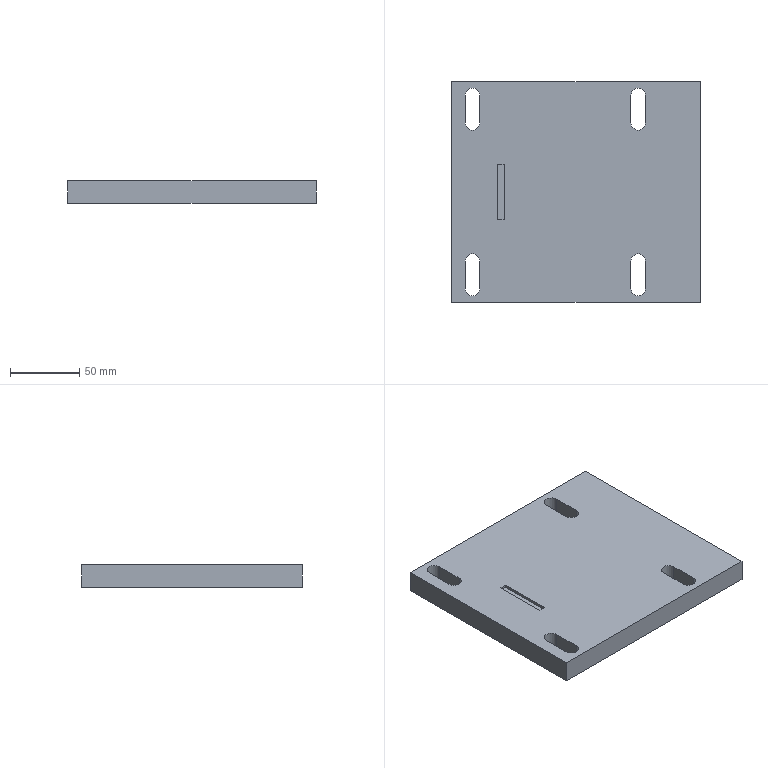Component | SolidWorks | CSFA2082 076-1 | 1 solid | 27 faces | box 180 x 160 x 16 mm | volume 441418 mm3 | plane 19 | cylinder 8 | commonest cylinder face diameters 10.5 x8
build123d program:
from build123d import *

# Parameters (mm, degrees)
SKETCH1_2_W              = 180
SKETCH1_2_H              = 160
EXTRUDE1_DEPTH           = 16
CUT_EXTRUDE1_DEPTH       = 122.474
SKETCH1_W                = 5
SKETCH1_H                = 40
SPRINGCORNERRELIEF_DEPTH = 2


with BuildPart() as part:
    # Sketch1_2 → Extrude1 (new body)
    with BuildSketch(Plane.XY):
        Rectangle(SKETCH1_2_W, SKETCH1_2_H)
    extrude(amount=EXTRUDE1_DEPTH)

    # Sketch2 → Cut-Extrude1 (cut, through all)
    with BuildSketch(Plane.XY.offset(16)):
        with BuildLine():
            Line((-69.75, 70), (-69.75, 50))
            ThreePointArc((-69.75, 50), (-75, 44.75), (-80.25, 50))
            Line((-80.25, 50), (-80.25, 70))
            ThreePointArc((-80.25, 70), (-75, 75.25), (-69.75, 70))
        make_face()
        with BuildLine():
            Line((-69.75, -50), (-69.75, -70))
            ThreePointArc((-69.75, -70), (-75, -75.25), (-80.25, -70))
            Line((-80.25, -70), (-80.25, -50))
            ThreePointArc((-80.25, -50), (-75, -44.75), (-69.75, -50))
        make_face()
        with BuildLine():
            Line((50.25, 70), (50.25, 50))
            ThreePointArc((50.25, 50), (45, 44.75), (39.75, 50))
            Line((39.75, 50), (39.75, 70))
            ThreePointArc((39.75, 70), (45, 75.25), (50.25, 70))
        make_face()
        with BuildLine():
            Line((50.25, -50), (50.25, -70))
            ThreePointArc((50.25, -70), (45, -75.25), (39.75, -70))
            Line((39.75, -70), (39.75, -50))
            ThreePointArc((39.75, -50), (45, -44.75), (50.25, -50))
        make_face()
    extrude(amount=-CUT_EXTRUDE1_DEPTH, mode=Mode.SUBTRACT)

    # Sketch1 → SpringCornerRelief (cut)
    with BuildSketch(Plane.XY.offset(16)):
        with Locations((-54.5, 0)):
            Rectangle(SKETCH1_W, SKETCH1_H)
    extrude(amount=-SPRINGCORNERRELIEF_DEPTH, mode=Mode.SUBTRACT)


solid = part.part

# Placed as in the assembly
solid = solid.moved(Location((187.301, -218.176, 657), (0, 0, 0)))
STEP:
#1=COLOUR_RGB('',0.7922,0.8196,0.9333);
#2=FILL_AREA_STYLE_COLOUR('',#1);
#3=FILL_AREA_STYLE('',(#2));
#4=SURFACE_STYLE_FILL_AREA(#3);
#5=SURFACE_SIDE_STYLE('',(#4));
#6=SURFACE_STYLE_USAGE(.BOTH.,#5);
#7=PRESENTATION_STYLE_ASSIGNMENT((#6));
#8=CARTESIAN_POINT('',(10.917,-11.739,25.866));
#9=VERTEX_POINT('',#8);
#10=CARTESIAN_POINT('',(10.917,-5.44,25.866));
#11=VERTEX_POINT('',#10);
#12=CARTESIAN_POINT('',(10.917,-11.739,25.866));
#13=DIRECTION('',(0.,1.,0.));
#14=VECTOR('',#13,39.37);
#15=LINE('',#12,#14);
#16=EDGE_CURVE('',#9,#11,#15,.T.);
#17=ORIENTED_EDGE('',*,*,#16,.T.);
#18=CARTESIAN_POINT('',(10.917,-5.44,26.496));
#19=VERTEX_POINT('',#18);
#20=CARTESIAN_POINT('',(10.917,-5.44,26.496));
#21=DIRECTION('',(0.,0.,-1.));
#22=VECTOR('',#21,39.37);
#23=LINE('',#20,#22);
#24=EDGE_CURVE('',#19,#11,#23,.T.);
#25=ORIENTED_EDGE('',*,*,#24,.F.);
#26=CARTESIAN_POINT('',(10.917,-11.739,26.496));
#27=VERTEX_POINT('',#26);
#28=CARTESIAN_POINT('',(10.917,-11.739,26.496));
#29=DIRECTION('',(0.,1.,0.));
#30=VECTOR('',#29,39.37);
#31=LINE('',#28,#30);
#32=EDGE_CURVE('',#27,#19,#31,.T.);
#33=ORIENTED_EDGE('',*,*,#32,.F.);
#34=CARTESIAN_POINT('',(10.917,-11.739,26.496));
#35=DIRECTION('',(0.,0.,-1.));
#36=VECTOR('',#35,39.37);
#37=LINE('',#34,#36);
#38=EDGE_CURVE('',#27,#9,#37,.T.);
#39=ORIENTED_EDGE('',*,*,#38,.T.);
#40=EDGE_LOOP('',(#17,#25,#33,#39));
#41=FACE_OUTER_BOUND('',#40,.T.);
#42=CARTESIAN_POINT('',(10.917,-11.739,26.496));
#43=DIRECTION('',(-1.,0.,0.));
#44=DIRECTION('',(0.,0.,1.));
#45=AXIS2_PLACEMENT_3D('',#42,#43,#44);
#46=PLANE('',#45);
#47=ADVANCED_FACE('',(#41),#46,.F.);
#48=CARTESIAN_POINT('',(3.831,-5.44,25.866));
#49=VERTEX_POINT('',#48);
#50=CARTESIAN_POINT('',(3.831,-5.44,25.866));
#51=DIRECTION('',(-1.,0.,0.));
#52=VECTOR('',#51,39.37);
#53=LINE('',#50,#52);
#54=EDGE_CURVE('',#11,#49,#53,.T.);
#55=ORIENTED_EDGE('',*,*,#54,.T.);
#56=CARTESIAN_POINT('',(3.831,-5.44,26.496));
#57=VERTEX_POINT('',#56);
#58=CARTESIAN_POINT('',(3.831,-5.44,26.496));
#59=DIRECTION('',(0.,0.,-1.));
#60=VECTOR('',#59,39.37);
#61=LINE('',#58,#60);
#62=EDGE_CURVE('',#57,#49,#61,.T.);
#63=ORIENTED_EDGE('',*,*,#62,.F.);
#64=CARTESIAN_POINT('',(3.831,-5.44,26.496));
#65=DIRECTION('',(-1.,0.,0.));
#66=VECTOR('',#65,39.37);
#67=LINE('',#64,#66);
#68=EDGE_CURVE('',#19,#57,#67,.T.);
#69=ORIENTED_EDGE('',*,*,#68,.F.);
#70=ORIENTED_EDGE('',*,*,#24,.T.);
#71=EDGE_LOOP('',(#55,#63,#69,#70));
#72=FACE_OUTER_BOUND('',#71,.T.);
#73=CARTESIAN_POINT('',(3.831,-5.44,26.496));
#74=DIRECTION('',(0.,-1.,0.));
#75=DIRECTION('',(0.,0.,-1.));
#76=AXIS2_PLACEMENT_3D('',#73,#74,#75);
#77=PLANE('',#76);
#78=ADVANCED_FACE('',(#72),#77,.F.);
#79=CARTESIAN_POINT('',(3.831,-11.739,25.866));
#80=VERTEX_POINT('',#79);
#81=CARTESIAN_POINT('',(3.831,-11.739,25.866));
#82=DIRECTION('',(0.,-1.,0.));
#83=VECTOR('',#82,39.37);
#84=LINE('',#81,#83);
#85=EDGE_CURVE('',#49,#80,#84,.T.);
#86=ORIENTED_EDGE('',*,*,#85,.T.);
#87=CARTESIAN_POINT('',(3.831,-11.739,26.496));
#88=VERTEX_POINT('',#87);
#89=CARTESIAN_POINT('',(3.831,-11.739,26.496));
#90=DIRECTION('',(0.,0.,-1.));
#91=VECTOR('',#90,39.37);
#92=LINE('',#89,#91);
#93=EDGE_CURVE('',#88,#80,#92,.T.);
#94=ORIENTED_EDGE('',*,*,#93,.F.);
#95=CARTESIAN_POINT('',(3.831,-11.739,26.496));
#96=DIRECTION('',(0.,-1.,0.));
#97=VECTOR('',#96,39.37);
#98=LINE('',#95,#97);
#99=EDGE_CURVE('',#57,#88,#98,.T.);
#100=ORIENTED_EDGE('',*,*,#99,.F.);
#101=ORIENTED_EDGE('',*,*,#62,.T.);
#102=EDGE_LOOP('',(#86,#94,#100,#101));
#103=FACE_OUTER_BOUND('',#102,.T.);
#104=CARTESIAN_POINT('',(3.831,-11.739,26.496));
#105=DIRECTION('',(1.,0.,0.));
#106=DIRECTION('',(0.,0.,-1.));
#107=AXIS2_PLACEMENT_3D('',#104,#105,#106);
#108=PLANE('',#107);
#109=ADVANCED_FACE('',(#103),#108,.F.);
#110=CARTESIAN_POINT('',(3.831,-11.739,25.866));
#111=DIRECTION('',(1.,0.,0.));
#112=VECTOR('',#111,39.37);
#113=LINE('',#110,#112);
#114=EDGE_CURVE('',#80,#9,#113,.T.);
#115=ORIENTED_EDGE('',*,*,#114,.T.);
#116=ORIENTED_EDGE('',*,*,#38,.F.);
#117=CARTESIAN_POINT('',(3.831,-11.739,26.496));
#118=DIRECTION('',(1.,0.,0.));
#119=VECTOR('',#118,39.37);
#120=LINE('',#117,#119);
#121=EDGE_CURVE('',#88,#27,#120,.T.);
#122=ORIENTED_EDGE('',*,*,#121,.F.);
#123=ORIENTED_EDGE('',*,*,#93,.T.);
#124=EDGE_LOOP('',(#115,#116,#122,#123));
#125=FACE_OUTER_BOUND('',#124,.T.);
#126=CARTESIAN_POINT('',(3.831,-11.739,26.496));
#127=DIRECTION('',(0.,1.,0.));
#128=DIRECTION('',(0.,0.,1.));
#129=AXIS2_PLACEMENT_3D('',#126,#127,#128);
#130=PLANE('',#129);
#131=ADVANCED_FACE('',(#125),#130,.F.);
#132=CARTESIAN_POINT('',(5.13,-9.377,26.496));
#133=VERTEX_POINT('',#132);
#134=CARTESIAN_POINT('',(5.327,-9.377,26.496));
#135=VERTEX_POINT('',#134);
#136=CARTESIAN_POINT('',(5.13,-9.377,26.496));
#137=DIRECTION('',(1.,0.,0.));
#138=VECTOR('',#137,39.37);
#139=LINE('',#136,#138);
#140=EDGE_CURVE('',#133,#135,#139,.T.);
#141=ORIENTED_EDGE('',*,*,#140,.F.);
#142=CARTESIAN_POINT('',(5.13,-7.802,26.496));
#143=VERTEX_POINT('',#142);
#144=CARTESIAN_POINT('',(5.13,-9.377,26.496));
#145=DIRECTION('',(0.,-1.,0.));
#146=VECTOR('',#145,39.37);
#147=LINE('',#144,#146);
#148=EDGE_CURVE('',#143,#133,#147,.T.);
#149=ORIENTED_EDGE('',*,*,#148,.F.);
#150=CARTESIAN_POINT('',(5.327,-7.802,26.496));
#151=VERTEX_POINT('',#150);
#152=CARTESIAN_POINT('',(5.13,-7.802,26.496));
#153=DIRECTION('',(-1.,0.,0.));
#154=VECTOR('',#153,39.37);
#155=LINE('',#152,#154);
#156=EDGE_CURVE('',#151,#143,#155,.T.);
#157=ORIENTED_EDGE('',*,*,#156,.F.);
#158=CARTESIAN_POINT('',(5.327,-9.377,26.496));
#159=DIRECTION('',(0.,1.,0.));
#160=VECTOR('',#159,39.37);
#161=LINE('',#158,#160);
#162=EDGE_CURVE('',#135,#151,#161,.T.);
#163=ORIENTED_EDGE('',*,*,#162,.F.);
#164=EDGE_LOOP('',(#141,#149,#157,#163));
#165=FACE_BOUND('',#164,.T.);
#166=CARTESIAN_POINT('',(8.939,-10.558,26.496));
#167=VERTEX_POINT('',#166);
#168=CARTESIAN_POINT('',(8.939,-11.346,26.496));
#169=VERTEX_POINT('',#168);
#170=CARTESIAN_POINT('',(8.939,-10.558,26.496));
#171=DIRECTION('',(0.,-1.,0.));
#172=VECTOR('',#171,39.37);
#173=LINE('',#170,#172);
#174=EDGE_CURVE('',#167,#169,#173,.T.);
#175=ORIENTED_EDGE('',*,*,#174,.F.);
#176=CARTESIAN_POINT('',(9.352,-10.558,26.496));
#177=VERTEX_POINT('',#176);
#178=CARTESIAN_POINT('',(9.146,-10.558,26.496));
#179=DIRECTION('',(0.,0.,1.));
#180=DIRECTION('',(1.,0.,0.));
#181=AXIS2_PLACEMENT_3D('',#178,#179,#180);
#182=CIRCLE('',#181,0.2067);
#183=EDGE_CURVE('',#177,#167,#182,.T.);
#184=ORIENTED_EDGE('',*,*,#183,.F.);
#185=CARTESIAN_POINT('',(9.352,-11.346,26.496));
#186=VERTEX_POINT('',#185);
#187=CARTESIAN_POINT('',(9.352,-10.558,26.496));
#188=DIRECTION('',(0.,1.,0.));
#189=VECTOR('',#188,39.37);
#190=LINE('',#187,#189);
#191=EDGE_CURVE('',#186,#177,#190,.T.);
#192=ORIENTED_EDGE('',*,*,#191,.F.);
#193=CARTESIAN_POINT('',(9.146,-11.346,26.496));
#194=DIRECTION('',(0.,0.,1.));
#195=DIRECTION('',(1.,0.,0.));
#196=AXIS2_PLACEMENT_3D('',#193,#194,#195);
#197=CIRCLE('',#196,0.2067);
#198=EDGE_CURVE('',#169,#186,#197,.T.);
#199=ORIENTED_EDGE('',*,*,#198,.F.);
#200=EDGE_LOOP('',(#175,#184,#192,#199));
#201=FACE_BOUND('',#200,.T.);
#202=CARTESIAN_POINT('',(8.939,-5.834,26.496));
#203=VERTEX_POINT('',#202);
#204=CARTESIAN_POINT('',(8.939,-6.621,26.496));
#205=VERTEX_POINT('',#204);
#206=CARTESIAN_POINT('',(8.939,-5.834,26.496));
#207=DIRECTION('',(0.,-1.,0.));
#208=VECTOR('',#207,39.37);
#209=LINE('',#206,#208);
#210=EDGE_CURVE('',#203,#205,#209,.T.);
#211=ORIENTED_EDGE('',*,*,#210,.F.);
#212=CARTESIAN_POINT('',(9.352,-5.834,26.496));
#213=VERTEX_POINT('',#212);
#214=CARTESIAN_POINT('',(9.146,-5.834,26.496));
#215=DIRECTION('',(0.,0.,1.));
#216=DIRECTION('',(1.,0.,0.));
#217=AXIS2_PLACEMENT_3D('',#214,#215,#216);
#218=CIRCLE('',#217,0.2067);
#219=EDGE_CURVE('',#213,#203,#218,.T.);
#220=ORIENTED_EDGE('',*,*,#219,.F.);
#221=CARTESIAN_POINT('',(9.352,-6.621,26.496));
#222=VERTEX_POINT('',#221);
#223=CARTESIAN_POINT('',(9.352,-5.834,26.496));
#224=DIRECTION('',(0.,1.,0.));
#225=VECTOR('',#224,39.37);
#226=LINE('',#223,#225);
#227=EDGE_CURVE('',#222,#213,#226,.T.);
#228=ORIENTED_EDGE('',*,*,#227,.F.);
#229=CARTESIAN_POINT('',(9.146,-6.621,26.496));
#230=DIRECTION('',(0.,0.,1.));
#231=DIRECTION('',(1.,0.,0.));
#232=AXIS2_PLACEMENT_3D('',#229,#230,#231);
#233=CIRCLE('',#232,0.2067);
#234=EDGE_CURVE('',#205,#222,#233,.T.);
#235=ORIENTED_EDGE('',*,*,#234,.F.);
#236=EDGE_LOOP('',(#211,#220,#228,#235));
#237=FACE_BOUND('',#236,.T.);
#238=CARTESIAN_POINT('',(4.215,-10.558,26.496));
#239=VERTEX_POINT('',#238);
#240=CARTESIAN_POINT('',(4.215,-11.346,26.496));
#241=VERTEX_POINT('',#240);
#242=CARTESIAN_POINT('',(4.215,-10.558,26.496));
#243=DIRECTION('',(0.,-1.,0.));
#244=VECTOR('',#243,39.37);
#245=LINE('',#242,#244);
#246=EDGE_CURVE('',#239,#241,#245,.T.);
#247=ORIENTED_EDGE('',*,*,#246,.F.);
#248=CARTESIAN_POINT('',(4.628,-10.558,26.496));
#249=VERTEX_POINT('',#248);
#250=CARTESIAN_POINT('',(4.421,-10.558,26.496));
#251=DIRECTION('',(0.,0.,1.));
#252=DIRECTION('',(1.,0.,0.));
#253=AXIS2_PLACEMENT_3D('',#250,#251,#252);
#254=CIRCLE('',#253,0.2067);
#255=EDGE_CURVE('',#249,#239,#254,.T.);
#256=ORIENTED_EDGE('',*,*,#255,.F.);
#257=CARTESIAN_POINT('',(4.628,-11.346,26.496));
#258=VERTEX_POINT('',#257);
#259=CARTESIAN_POINT('',(4.628,-10.558,26.496));
#260=DIRECTION('',(0.,1.,0.));
#261=VECTOR('',#260,39.37);
#262=LINE('',#259,#261);
#263=EDGE_CURVE('',#258,#249,#262,.T.);
#264=ORIENTED_EDGE('',*,*,#263,.F.);
#265=CARTESIAN_POINT('',(4.421,-11.346,26.496));
#266=DIRECTION('',(0.,0.,1.));
#267=DIRECTION('',(1.,0.,0.));
#268=AXIS2_PLACEMENT_3D('',#265,#266,#267);
#269=CIRCLE('',#268,0.2067);
#270=EDGE_CURVE('',#241,#258,#269,.T.);
#271=ORIENTED_EDGE('',*,*,#270,.F.);
#272=EDGE_LOOP('',(#247,#256,#264,#271));
#273=FACE_BOUND('',#272,.T.);
#274=CARTESIAN_POINT('',(4.215,-5.834,26.496));
#275=VERTEX_POINT('',#274);
#276=CARTESIAN_POINT('',(4.215,-6.621,26.496));
#277=VERTEX_POINT('',#276);
#278=CARTESIAN_POINT('',(4.215,-5.834,26.496));
#279=DIRECTION('',(0.,-1.,0.));
#280=VECTOR('',#279,39.37);
#281=LINE('',#278,#280);
#282=EDGE_CURVE('',#275,#277,#281,.T.);
#283=ORIENTED_EDGE('',*,*,#282,.F.);
#284=CARTESIAN_POINT('',(4.628,-5.834,26.496));
#285=VERTEX_POINT('',#284);
#286=CARTESIAN_POINT('',(4.421,-5.834,26.496));
#287=DIRECTION('',(0.,0.,1.));
#288=DIRECTION('',(1.,0.,0.));
#289=AXIS2_PLACEMENT_3D('',#286,#287,#288);
#290=CIRCLE('',#289,0.2067);
#291=EDGE_CURVE('',#285,#275,#290,.T.);
#292=ORIENTED_EDGE('',*,*,#291,.F.);
#293=CARTESIAN_POINT('',(4.628,-6.621,26.496));
#294=VERTEX_POINT('',#293);
#295=CARTESIAN_POINT('',(4.628,-5.834,26.496));
#296=DIRECTION('',(0.,1.,0.));
#297=VECTOR('',#296,39.37);
#298=LINE('',#295,#297);
#299=EDGE_CURVE('',#294,#285,#298,.T.);
#300=ORIENTED_EDGE('',*,*,#299,.F.);
#301=CARTESIAN_POINT('',(4.421,-6.621,26.496));
#302=DIRECTION('',(0.,0.,1.));
#303=DIRECTION('',(1.,0.,0.));
#304=AXIS2_PLACEMENT_3D('',#301,#302,#303);
#305=CIRCLE('',#304,0.2067);
#306=EDGE_CURVE('',#277,#294,#305,.T.);
#307=ORIENTED_EDGE('',*,*,#306,.F.);
#308=EDGE_LOOP('',(#283,#292,#300,#307));
#309=FACE_BOUND('',#308,.T.);
#310=ORIENTED_EDGE('',*,*,#32,.T.);
#311=ORIENTED_EDGE('',*,*,#68,.T.);
#312=ORIENTED_EDGE('',*,*,#99,.T.);
#313=ORIENTED_EDGE('',*,*,#121,.T.);
#314=EDGE_LOOP('',(#310,#311,#312,#313));
#315=FACE_OUTER_BOUND('',#314,.T.);
#316=CARTESIAN_POINT('',(10.917,-5.44,26.496));
#317=DIRECTION('',(0.,0.,-1.));
#318=DIRECTION('',(-1.,0.,0.));
#319=AXIS2_PLACEMENT_3D('',#316,#317,#318);
#320=PLANE('',#319);
#321=ADVANCED_FACE('',(#165,#201,#237,#273,#309,#315),#320,.F.);
#322=CARTESIAN_POINT('',(9.352,-10.558,25.866));
#323=VERTEX_POINT('',#322);
#324=CARTESIAN_POINT('',(8.939,-10.558,25.866));
#325=VERTEX_POINT('',#324);
#326=CARTESIAN_POINT('',(9.146,-10.558,25.866));
#327=DIRECTION('',(0.,0.,1.));
#328=DIRECTION('',(1.,0.,0.));
#329=AXIS2_PLACEMENT_3D('',#326,#327,#328);
#330=CIRCLE('',#329,0.2067);
#331=EDGE_CURVE('',#323,#325,#330,.T.);
#332=ORIENTED_EDGE('',*,*,#331,.T.);
#333=CARTESIAN_POINT('',(8.939,-11.346,25.866));
#334=VERTEX_POINT('',#333);
#335=CARTESIAN_POINT('',(8.939,-10.558,25.866));
#336=DIRECTION('',(0.,-1.,0.));
#337=VECTOR('',#336,39.37);
#338=LINE('',#335,#337);
#339=EDGE_CURVE('',#325,#334,#338,.T.);
#340=ORIENTED_EDGE('',*,*,#339,.T.);
#341=CARTESIAN_POINT('',(9.352,-11.346,25.866));
#342=VERTEX_POINT('',#341);
#343=CARTESIAN_POINT('',(9.146,-11.346,25.866));
#344=DIRECTION('',(0.,0.,1.));
#345=DIRECTION('',(1.,0.,0.));
#346=AXIS2_PLACEMENT_3D('',#343,#344,#345);
#347=CIRCLE('',#346,0.2067);
#348=EDGE_CURVE('',#334,#342,#347,.T.);
#349=ORIENTED_EDGE('',*,*,#348,.T.);
#350=CARTESIAN_POINT('',(9.352,-10.558,25.866));
#351=DIRECTION('',(0.,1.,0.));
#352=VECTOR('',#351,39.37);
#353=LINE('',#350,#352);
#354=EDGE_CURVE('',#342,#323,#353,.T.);
#355=ORIENTED_EDGE('',*,*,#354,.T.);
#356=EDGE_LOOP('',(#332,#340,#349,#355));
#357=FACE_BOUND('',#356,.T.);
#358=CARTESIAN_POINT('',(9.352,-5.834,25.866));
#359=VERTEX_POINT('',#358);
#360=CARTESIAN_POINT('',(8.939,-5.834,25.866));
#361=VERTEX_POINT('',#360);
#362=CARTESIAN_POINT('',(9.146,-5.834,25.866));
#363=DIRECTION('',(0.,0.,1.));
#364=DIRECTION('',(1.,0.,0.));
#365=AXIS2_PLACEMENT_3D('',#362,#363,#364);
#366=CIRCLE('',#365,0.2067);
#367=EDGE_CURVE('',#359,#361,#366,.T.);
#368=ORIENTED_EDGE('',*,*,#367,.T.);
#369=CARTESIAN_POINT('',(8.939,-6.621,25.866));
#370=VERTEX_POINT('',#369);
#371=CARTESIAN_POINT('',(8.939,-5.834,25.866));
#372=DIRECTION('',(0.,-1.,0.));
#373=VECTOR('',#372,39.37);
#374=LINE('',#371,#373);
#375=EDGE_CURVE('',#361,#370,#374,.T.);
#376=ORIENTED_EDGE('',*,*,#375,.T.);
#377=CARTESIAN_POINT('',(9.352,-6.621,25.866));
#378=VERTEX_POINT('',#377);
#379=CARTESIAN_POINT('',(9.146,-6.621,25.866));
#380=DIRECTION('',(0.,0.,1.));
#381=DIRECTION('',(1.,0.,0.));
#382=AXIS2_PLACEMENT_3D('',#379,#380,#381);
#383=CIRCLE('',#382,0.2067);
#384=EDGE_CURVE('',#370,#378,#383,.T.);
#385=ORIENTED_EDGE('',*,*,#384,.T.);
#386=CARTESIAN_POINT('',(9.352,-5.834,25.866));
#387=DIRECTION('',(0.,1.,0.));
#388=VECTOR('',#387,39.37);
#389=LINE('',#386,#388);
#390=EDGE_CURVE('',#378,#359,#389,.T.);
#391=ORIENTED_EDGE('',*,*,#390,.T.);
#392=EDGE_LOOP('',(#368,#376,#385,#391));
#393=FACE_BOUND('',#392,.T.);
#394=CARTESIAN_POINT('',(4.628,-10.558,25.866));
#395=VERTEX_POINT('',#394);
#396=CARTESIAN_POINT('',(4.215,-10.558,25.866));
#397=VERTEX_POINT('',#396);
#398=CARTESIAN_POINT('',(4.421,-10.558,25.866));
#399=DIRECTION('',(0.,0.,1.));
#400=DIRECTION('',(1.,0.,0.));
#401=AXIS2_PLACEMENT_3D('',#398,#399,#400);
#402=CIRCLE('',#401,0.2067);
#403=EDGE_CURVE('',#395,#397,#402,.T.);
#404=ORIENTED_EDGE('',*,*,#403,.T.);
#405=CARTESIAN_POINT('',(4.215,-11.346,25.866));
#406=VERTEX_POINT('',#405);
#407=CARTESIAN_POINT('',(4.215,-10.558,25.866));
#408=DIRECTION('',(0.,-1.,0.));
#409=VECTOR('',#408,39.37);
#410=LINE('',#407,#409);
#411=EDGE_CURVE('',#397,#406,#410,.T.);
#412=ORIENTED_EDGE('',*,*,#411,.T.);
#413=CARTESIAN_POINT('',(4.628,-11.346,25.866));
#414=VERTEX_POINT('',#413);
#415=CARTESIAN_POINT('',(4.421,-11.346,25.866));
#416=DIRECTION('',(0.,0.,1.));
#417=DIRECTION('',(1.,0.,0.));
#418=AXIS2_PLACEMENT_3D('',#415,#416,#417);
#419=CIRCLE('',#418,0.2067);
#420=EDGE_CURVE('',#406,#414,#419,.T.);
#421=ORIENTED_EDGE('',*,*,#420,.T.);
#422=CARTESIAN_POINT('',(4.628,-10.558,25.866));
#423=DIRECTION('',(0.,1.,0.));
#424=VECTOR('',#423,39.37);
#425=LINE('',#422,#424);
#426=EDGE_CURVE('',#414,#395,#425,.T.);
#427=ORIENTED_EDGE('',*,*,#426,.T.);
#428=EDGE_LOOP('',(#404,#412,#421,#427));
#429=FACE_BOUND('',#428,.T.);
#430=CARTESIAN_POINT('',(4.628,-5.834,25.866));
#431=VERTEX_POINT('',#430);
#432=CARTESIAN_POINT('',(4.215,-5.834,25.866));
#433=VERTEX_POINT('',#432);
#434=CARTESIAN_POINT('',(4.421,-5.834,25.866));
#435=DIRECTION('',(0.,0.,1.));
#436=DIRECTION('',(1.,0.,0.));
#437=AXIS2_PLACEMENT_3D('',#434,#435,#436);
#438=CIRCLE('',#437,0.2067);
#439=EDGE_CURVE('',#431,#433,#438,.T.);
#440=ORIENTED_EDGE('',*,*,#439,.T.);
#441=CARTESIAN_POINT('',(4.215,-6.621,25.866));
#442=VERTEX_POINT('',#441);
#443=CARTESIAN_POINT('',(4.215,-5.834,25.866));
#444=DIRECTION('',(0.,-1.,0.));
#445=VECTOR('',#444,39.37);
#446=LINE('',#443,#445);
#447=EDGE_CURVE('',#433,#442,#446,.T.);
#448=ORIENTED_EDGE('',*,*,#447,.T.);
#449=CARTESIAN_POINT('',(4.628,-6.621,25.866));
#450=VERTEX_POINT('',#449);
#451=CARTESIAN_POINT('',(4.421,-6.621,25.866));
#452=DIRECTION('',(0.,0.,1.));
#453=DIRECTION('',(1.,0.,0.));
#454=AXIS2_PLACEMENT_3D('',#451,#452,#453);
#455=CIRCLE('',#454,0.2067);
#456=EDGE_CURVE('',#442,#450,#455,.T.);
#457=ORIENTED_EDGE('',*,*,#456,.T.);
#458=CARTESIAN_POINT('',(4.628,-5.834,25.866));
#459=DIRECTION('',(0.,1.,0.));
#460=VECTOR('',#459,39.37);
#461=LINE('',#458,#460);
#462=EDGE_CURVE('',#450,#431,#461,.T.);
#463=ORIENTED_EDGE('',*,*,#462,.T.);
#464=EDGE_LOOP('',(#440,#448,#457,#463));
#465=FACE_BOUND('',#464,.T.);
#466=ORIENTED_EDGE('',*,*,#16,.F.);
#467=ORIENTED_EDGE('',*,*,#114,.F.);
#468=ORIENTED_EDGE('',*,*,#85,.F.);
#469=ORIENTED_EDGE('',*,*,#54,.F.);
#470=EDGE_LOOP('',(#466,#467,#468,#469));
#471=FACE_OUTER_BOUND('',#470,.T.);
#472=CARTESIAN_POINT('',(10.917,-5.44,25.866));
#473=DIRECTION('',(0.,0.,-1.));
#474=DIRECTION('',(-1.,0.,0.));
#475=AXIS2_PLACEMENT_3D('',#472,#473,#474);
#476=PLANE('',#475);
#477=ADVANCED_FACE('',(#357,#393,#429,#465,#471),#476,.T.);
#478=ORIENTED_EDGE('',*,*,#291,.T.);
#479=CARTESIAN_POINT('',(4.215,-5.834,25.866));
#480=DIRECTION('',(0.,0.,1.));
#481=VECTOR('',#480,39.37);
#482=LINE('',#479,#481);
#483=EDGE_CURVE('',#433,#275,#482,.T.);
#484=ORIENTED_EDGE('',*,*,#483,.F.);
#485=ORIENTED_EDGE('',*,*,#439,.F.);
#486=CARTESIAN_POINT('',(4.628,-5.834,25.866));
#487=DIRECTION('',(0.,0.,1.));
#488=VECTOR('',#487,39.37);
#489=LINE('',#486,#488);
#490=EDGE_CURVE('',#431,#285,#489,.T.);
#491=ORIENTED_EDGE('',*,*,#490,.T.);
#492=EDGE_LOOP('',(#478,#484,#485,#491));
#493=FACE_OUTER_BOUND('',#492,.T.);
#494=CARTESIAN_POINT('',(4.421,-5.834,25.866));
#495=DIRECTION('',(0.,0.,1.));
#496=DIRECTION('',(1.,0.,0.));
#497=AXIS2_PLACEMENT_3D('',#494,#495,#496);
#498=CYLINDRICAL_SURFACE('',#497,0.2067);
#499=ADVANCED_FACE('',(#493),#498,.F.);
#500=ORIENTED_EDGE('',*,*,#299,.T.);
#501=ORIENTED_EDGE('',*,*,#490,.F.);
#502=ORIENTED_EDGE('',*,*,#462,.F.);
#503=CARTESIAN_POINT('',(4.628,-6.621,25.866));
#504=DIRECTION('',(0.,0.,1.));
#505=VECTOR('',#504,39.37);
#506=LINE('',#503,#505);
#507=EDGE_CURVE('',#450,#294,#506,.T.);
#508=ORIENTED_EDGE('',*,*,#507,.T.);
#509=EDGE_LOOP('',(#500,#501,#502,#508));
#510=FACE_OUTER_BOUND('',#509,.T.);
#511=CARTESIAN_POINT('',(4.628,-5.834,25.866));
#512=DIRECTION('',(1.,0.,0.));
#513=DIRECTION('',(0.,0.,-1.));
#514=AXIS2_PLACEMENT_3D('',#511,#512,#513);
#515=PLANE('',#514);
#516=ADVANCED_FACE('',(#510),#515,.F.);
#517=ORIENTED_EDGE('',*,*,#306,.T.);
#518=ORIENTED_EDGE('',*,*,#507,.F.);
#519=ORIENTED_EDGE('',*,*,#456,.F.);
#520=CARTESIAN_POINT('',(4.215,-6.621,25.866));
#521=DIRECTION('',(0.,0.,1.));
#522=VECTOR('',#521,39.37);
#523=LINE('',#520,#522);
#524=EDGE_CURVE('',#442,#277,#523,.T.);
#525=ORIENTED_EDGE('',*,*,#524,.T.);
#526=EDGE_LOOP('',(#517,#518,#519,#525));
#527=FACE_OUTER_BOUND('',#526,.T.);
#528=CARTESIAN_POINT('',(4.421,-6.621,25.866));
#529=DIRECTION('',(0.,0.,1.));
#530=DIRECTION('',(1.,0.,0.));
#531=AXIS2_PLACEMENT_3D('',#528,#529,#530);
#532=CYLINDRICAL_SURFACE('',#531,0.2067);
#533=ADVANCED_FACE('',(#527),#532,.F.);
#534=ORIENTED_EDGE('',*,*,#282,.T.);
#535=ORIENTED_EDGE('',*,*,#524,.F.);
#536=ORIENTED_EDGE('',*,*,#447,.F.);
#537=ORIENTED_EDGE('',*,*,#483,.T.);
#538=EDGE_LOOP('',(#534,#535,#536,#537));
#539=FACE_OUTER_BOUND('',#538,.T.);
#540=CARTESIAN_POINT('',(4.215,-5.834,25.866));
#541=DIRECTION('',(-1.,0.,0.));
#542=DIRECTION('',(0.,0.,1.));
#543=AXIS2_PLACEMENT_3D('',#540,#541,#542);
#544=PLANE('',#543);
#545=ADVANCED_FACE('',(#539),#544,.F.);
#546=ORIENTED_EDGE('',*,*,#255,.T.);
#547=CARTESIAN_POINT('',(4.215,-10.558,25.866));
#548=DIRECTION('',(0.,0.,1.));
#549=VECTOR('',#548,39.37);
#550=LINE('',#547,#549);
#551=EDGE_CURVE('',#397,#239,#550,.T.);
#552=ORIENTED_EDGE('',*,*,#551,.F.);
#553=ORIENTED_EDGE('',*,*,#403,.F.);
#554=CARTESIAN_POINT('',(4.628,-10.558,25.866));
#555=DIRECTION('',(0.,0.,1.));
#556=VECTOR('',#555,39.37);
#557=LINE('',#554,#556);
#558=EDGE_CURVE('',#395,#249,#557,.T.);
#559=ORIENTED_EDGE('',*,*,#558,.T.);
#560=EDGE_LOOP('',(#546,#552,#553,#559));
#561=FACE_OUTER_BOUND('',#560,.T.);
#562=CARTESIAN_POINT('',(4.421,-10.558,25.866));
#563=DIRECTION('',(0.,0.,1.));
#564=DIRECTION('',(1.,0.,0.));
#565=AXIS2_PLACEMENT_3D('',#562,#563,#564);
#566=CYLINDRICAL_SURFACE('',#565,0.2067);
#567=ADVANCED_FACE('',(#561),#566,.F.);
#568=ORIENTED_EDGE('',*,*,#263,.T.);
#569=ORIENTED_EDGE('',*,*,#558,.F.);
#570=ORIENTED_EDGE('',*,*,#426,.F.);
#571=CARTESIAN_POINT('',(4.628,-11.346,25.866));
#572=DIRECTION('',(0.,0.,1.));
#573=VECTOR('',#572,39.37);
#574=LINE('',#571,#573);
#575=EDGE_CURVE('',#414,#258,#574,.T.);
#576=ORIENTED_EDGE('',*,*,#575,.T.);
#577=EDGE_LOOP('',(#568,#569,#570,#576));
#578=FACE_OUTER_BOUND('',#577,.T.);
#579=CARTESIAN_POINT('',(4.628,-10.558,25.866));
#580=DIRECTION('',(1.,0.,0.));
#581=DIRECTION('',(0.,0.,-1.));
#582=AXIS2_PLACEMENT_3D('',#579,#580,#581);
#583=PLANE('',#582);
#584=ADVANCED_FACE('',(#578),#583,.F.);
#585=ORIENTED_EDGE('',*,*,#270,.T.);
#586=ORIENTED_EDGE('',*,*,#575,.F.);
#587=ORIENTED_EDGE('',*,*,#420,.F.);
#588=CARTESIAN_POINT('',(4.215,-11.346,25.866));
#589=DIRECTION('',(0.,0.,1.));
#590=VECTOR('',#589,39.37);
#591=LINE('',#588,#590);
#592=EDGE_CURVE('',#406,#241,#591,.T.);
#593=ORIENTED_EDGE('',*,*,#592,.T.);
#594=EDGE_LOOP('',(#585,#586,#587,#593));
#595=FACE_OUTER_BOUND('',#594,.T.);
#596=CARTESIAN_POINT('',(4.421,-11.346,25.866));
#597=DIRECTION('',(0.,0.,1.));
#598=DIRECTION('',(1.,0.,0.));
#599=AXIS2_PLACEMENT_3D('',#596,#597,#598);
#600=CYLINDRICAL_SURFACE('',#599,0.2067);
#601=ADVANCED_FACE('',(#595),#600,.F.);
#602=ORIENTED_EDGE('',*,*,#246,.T.);
#603=ORIENTED_EDGE('',*,*,#592,.F.);
#604=ORIENTED_EDGE('',*,*,#411,.F.);
#605=ORIENTED_EDGE('',*,*,#551,.T.);
#606=EDGE_LOOP('',(#602,#603,#604,#605));
#607=FACE_OUTER_BOUND('',#606,.T.);
#608=CARTESIAN_POINT('',(4.215,-10.558,25.866));
#609=DIRECTION('',(-1.,0.,0.));
#610=DIRECTION('',(0.,0.,1.));
#611=AXIS2_PLACEMENT_3D('',#608,#609,#610);
#612=PLANE('',#611);
#613=ADVANCED_FACE('',(#607),#612,.F.);
#614=ORIENTED_EDGE('',*,*,#219,.T.);
#615=CARTESIAN_POINT('',(8.939,-5.834,25.866));
#616=DIRECTION('',(0.,0.,1.));
#617=VECTOR('',#616,39.37);
#618=LINE('',#615,#617);
#619=EDGE_CURVE('',#361,#203,#618,.T.);
#620=ORIENTED_EDGE('',*,*,#619,.F.);
#621=ORIENTED_EDGE('',*,*,#367,.F.);
#622=CARTESIAN_POINT('',(9.352,-5.834,25.866));
#623=DIRECTION('',(0.,0.,1.));
#624=VECTOR('',#623,39.37);
#625=LINE('',#622,#624);
#626=EDGE_CURVE('',#359,#213,#625,.T.);
#627=ORIENTED_EDGE('',*,*,#626,.T.);
#628=EDGE_LOOP('',(#614,#620,#621,#627));
#629=FACE_OUTER_BOUND('',#628,.T.);
#630=CARTESIAN_POINT('',(9.146,-5.834,25.866));
#631=DIRECTION('',(0.,0.,1.));
#632=DIRECTION('',(1.,0.,0.));
#633=AXIS2_PLACEMENT_3D('',#630,#631,#632);
#634=CYLINDRICAL_SURFACE('',#633,0.2067);
#635=ADVANCED_FACE('',(#629),#634,.F.);
#636=ORIENTED_EDGE('',*,*,#227,.T.);
#637=ORIENTED_EDGE('',*,*,#626,.F.);
#638=ORIENTED_EDGE('',*,*,#390,.F.);
#639=CARTESIAN_POINT('',(9.352,-6.621,25.866));
#640=DIRECTION('',(0.,0.,1.));
#641=VECTOR('',#640,39.37);
#642=LINE('',#639,#641);
#643=EDGE_CURVE('',#378,#222,#642,.T.);
#644=ORIENTED_EDGE('',*,*,#643,.T.);
#645=EDGE_LOOP('',(#636,#637,#638,#644));
#646=FACE_OUTER_BOUND('',#645,.T.);
#647=CARTESIAN_POINT('',(9.352,-5.834,25.866));
#648=DIRECTION('',(1.,0.,0.));
#649=DIRECTION('',(0.,0.,-1.));
#650=AXIS2_PLACEMENT_3D('',#647,#648,#649);
#651=PLANE('',#650);
#652=ADVANCED_FACE('',(#646),#651,.F.);
#653=ORIENTED_EDGE('',*,*,#234,.T.);
#654=ORIENTED_EDGE('',*,*,#643,.F.);
#655=ORIENTED_EDGE('',*,*,#384,.F.);
#656=CARTESIAN_POINT('',(8.939,-6.621,25.866));
#657=DIRECTION('',(0.,0.,1.));
#658=VECTOR('',#657,39.37);
#659=LINE('',#656,#658);
#660=EDGE_CURVE('',#370,#205,#659,.T.);
#661=ORIENTED_EDGE('',*,*,#660,.T.);
#662=EDGE_LOOP('',(#653,#654,#655,#661));
#663=FACE_OUTER_BOUND('',#662,.T.);
#664=CARTESIAN_POINT('',(9.146,-6.621,25.866));
#665=DIRECTION('',(0.,0.,1.));
#666=DIRECTION('',(1.,0.,0.));
#667=AXIS2_PLACEMENT_3D('',#664,#665,#666);
#668=CYLINDRICAL_SURFACE('',#667,0.2067);
#669=ADVANCED_FACE('',(#663),#668,.F.);
#670=ORIENTED_EDGE('',*,*,#210,.T.);
#671=ORIENTED_EDGE('',*,*,#660,.F.);
#672=ORIENTED_EDGE('',*,*,#375,.F.);
#673=ORIENTED_EDGE('',*,*,#619,.T.);
#674=EDGE_LOOP('',(#670,#671,#672,#673));
#675=FACE_OUTER_BOUND('',#674,.T.);
#676=CARTESIAN_POINT('',(8.939,-5.834,25.866));
#677=DIRECTION('',(-1.,0.,0.));
#678=DIRECTION('',(0.,0.,1.));
#679=AXIS2_PLACEMENT_3D('',#676,#677,#678);
#680=PLANE('',#679);
#681=ADVANCED_FACE('',(#675),#680,.F.);
#682=ORIENTED_EDGE('',*,*,#183,.T.);
#683=CARTESIAN_POINT('',(8.939,-10.558,25.866));
#684=DIRECTION('',(0.,0.,1.));
#685=VECTOR('',#684,39.37);
#686=LINE('',#683,#685);
#687=EDGE_CURVE('',#325,#167,#686,.T.);
#688=ORIENTED_EDGE('',*,*,#687,.F.);
#689=ORIENTED_EDGE('',*,*,#331,.F.);
#690=CARTESIAN_POINT('',(9.352,-10.558,25.866));
#691=DIRECTION('',(0.,0.,1.));
#692=VECTOR('',#691,39.37);
#693=LINE('',#690,#692);
#694=EDGE_CURVE('',#323,#177,#693,.T.);
#695=ORIENTED_EDGE('',*,*,#694,.T.);
#696=EDGE_LOOP('',(#682,#688,#689,#695));
#697=FACE_OUTER_BOUND('',#696,.T.);
#698=CARTESIAN_POINT('',(9.146,-10.558,25.866));
#699=DIRECTION('',(0.,0.,1.));
#700=DIRECTION('',(1.,0.,0.));
#701=AXIS2_PLACEMENT_3D('',#698,#699,#700);
#702=CYLINDRICAL_SURFACE('',#701,0.2067);
#703=ADVANCED_FACE('',(#697),#702,.F.);
#704=ORIENTED_EDGE('',*,*,#191,.T.);
#705=ORIENTED_EDGE('',*,*,#694,.F.);
#706=ORIENTED_EDGE('',*,*,#354,.F.);
#707=CARTESIAN_POINT('',(9.352,-11.346,25.866));
#708=DIRECTION('',(0.,0.,1.));
#709=VECTOR('',#708,39.37);
#710=LINE('',#707,#709);
#711=EDGE_CURVE('',#342,#186,#710,.T.);
#712=ORIENTED_EDGE('',*,*,#711,.T.);
#713=EDGE_LOOP('',(#704,#705,#706,#712));
#714=FACE_OUTER_BOUND('',#713,.T.);
#715=CARTESIAN_POINT('',(9.352,-10.558,25.866));
#716=DIRECTION('',(1.,0.,0.));
#717=DIRECTION('',(0.,0.,-1.));
#718=AXIS2_PLACEMENT_3D('',#715,#716,#717);
#719=PLANE('',#718);
#720=ADVANCED_FACE('',(#714),#719,.F.);
#721=ORIENTED_EDGE('',*,*,#198,.T.);
#722=ORIENTED_EDGE('',*,*,#711,.F.);
#723=ORIENTED_EDGE('',*,*,#348,.F.);
#724=CARTESIAN_POINT('',(8.939,-11.346,25.866));
#725=DIRECTION('',(0.,0.,1.));
#726=VECTOR('',#725,39.37);
#727=LINE('',#724,#726);
#728=EDGE_CURVE('',#334,#169,#727,.T.);
#729=ORIENTED_EDGE('',*,*,#728,.T.);
#730=EDGE_LOOP('',(#721,#722,#723,#729));
#731=FACE_OUTER_BOUND('',#730,.T.);
#732=CARTESIAN_POINT('',(9.146,-11.346,25.866));
#733=DIRECTION('',(0.,0.,1.));
#734=DIRECTION('',(1.,0.,0.));
#735=AXIS2_PLACEMENT_3D('',#732,#733,#734);
#736=CYLINDRICAL_SURFACE('',#735,0.2067);
#737=ADVANCED_FACE('',(#731),#736,.F.);
#738=ORIENTED_EDGE('',*,*,#174,.T.);
#739=ORIENTED_EDGE('',*,*,#728,.F.);
#740=ORIENTED_EDGE('',*,*,#339,.F.);
#741=ORIENTED_EDGE('',*,*,#687,.T.);
#742=EDGE_LOOP('',(#738,#739,#740,#741));
#743=FACE_OUTER_BOUND('',#742,.T.);
#744=CARTESIAN_POINT('',(8.939,-10.558,25.866));
#745=DIRECTION('',(-1.,0.,0.));
#746=DIRECTION('',(0.,0.,1.));
#747=AXIS2_PLACEMENT_3D('',#744,#745,#746);
#748=PLANE('',#747);
#749=ADVANCED_FACE('',(#743),#748,.F.);
#750=ORIENTED_EDGE('',*,*,#148,.T.);
#751=CARTESIAN_POINT('',(5.13,-9.377,26.417));
#752=VERTEX_POINT('',#751);
#753=CARTESIAN_POINT('',(5.13,-9.377,26.417));
#754=DIRECTION('',(0.,0.,1.));
#755=VECTOR('',#754,39.37);
#756=LINE('',#753,#755);
#757=EDGE_CURVE('',#752,#133,#756,.T.);
#758=ORIENTED_EDGE('',*,*,#757,.F.);
#759=CARTESIAN_POINT('',(5.13,-7.802,26.417));
#760=VERTEX_POINT('',#759);
#761=CARTESIAN_POINT('',(5.13,-9.377,26.417));
#762=DIRECTION('',(0.,-1.,0.));
#763=VECTOR('',#762,39.37);
#764=LINE('',#761,#763);
#765=EDGE_CURVE('',#760,#752,#764,.T.);
#766=ORIENTED_EDGE('',*,*,#765,.F.);
#767=CARTESIAN_POINT('',(5.13,-7.802,26.417));
#768=DIRECTION('',(0.,0.,1.));
#769=VECTOR('',#768,39.37);
#770=LINE('',#767,#769);
#771=EDGE_CURVE('',#760,#143,#770,.T.);
#772=ORIENTED_EDGE('',*,*,#771,.T.);
#773=EDGE_LOOP('',(#750,#758,#766,#772));
#774=FACE_OUTER_BOUND('',#773,.T.);
#775=CARTESIAN_POINT('',(5.13,-9.377,26.417));
#776=DIRECTION('',(-1.,0.,0.));
#777=DIRECTION('',(0.,0.,1.));
#778=AXIS2_PLACEMENT_3D('',#775,#776,#777);
#779=PLANE('',#778);
#780=ADVANCED_FACE('',(#774),#779,.F.);
#781=ORIENTED_EDGE('',*,*,#156,.T.);
#782=ORIENTED_EDGE('',*,*,#771,.F.);
#783=CARTESIAN_POINT('',(5.327,-7.802,26.417));
#784=VERTEX_POINT('',#783);
#785=CARTESIAN_POINT('',(5.13,-7.802,26.417));
#786=DIRECTION('',(-1.,0.,0.));
#787=VECTOR('',#786,39.37);
#788=LINE('',#785,#787);
#789=EDGE_CURVE('',#784,#760,#788,.T.);
#790=ORIENTED_EDGE('',*,*,#789,.F.);
#791=CARTESIAN_POINT('',(5.327,-7.802,26.417));
#792=DIRECTION('',(0.,0.,1.));
#793=VECTOR('',#792,39.37);
#794=LINE('',#791,#793);
#795=EDGE_CURVE('',#784,#151,#794,.T.);
#796=ORIENTED_EDGE('',*,*,#795,.T.);
#797=EDGE_LOOP('',(#781,#782,#790,#796));
#798=FACE_OUTER_BOUND('',#797,.T.);
#799=CARTESIAN_POINT('',(5.13,-7.802,26.417));
#800=DIRECTION('',(0.,1.,0.));
#801=DIRECTION('',(0.,0.,1.));
#802=AXIS2_PLACEMENT_3D('',#799,#800,#801);
#803=PLANE('',#802);
#804=ADVANCED_FACE('',(#798),#803,.F.);
#805=ORIENTED_EDGE('',*,*,#162,.T.);
#806=ORIENTED_EDGE('',*,*,#795,.F.);
#807=CARTESIAN_POINT('',(5.327,-9.377,26.417));
#808=VERTEX_POINT('',#807);
#809=CARTESIAN_POINT('',(5.327,-9.377,26.417));
#810=DIRECTION('',(0.,1.,0.));
#811=VECTOR('',#810,39.37);
#812=LINE('',#809,#811);
#813=EDGE_CURVE('',#808,#784,#812,.T.);
#814=ORIENTED_EDGE('',*,*,#813,.F.);
#815=CARTESIAN_POINT('',(5.327,-9.377,26.417));
#816=DIRECTION('',(0.,0.,1.));
#817=VECTOR('',#816,39.37);
#818=LINE('',#815,#817);
#819=EDGE_CURVE('',#808,#135,#818,.T.);
#820=ORIENTED_EDGE('',*,*,#819,.T.);
#821=EDGE_LOOP('',(#805,#806,#814,#820));
#822=FACE_OUTER_BOUND('',#821,.T.);
#823=CARTESIAN_POINT('',(5.327,-9.377,26.417));
#824=DIRECTION('',(1.,0.,0.));
#825=DIRECTION('',(0.,0.,-1.));
#826=AXIS2_PLACEMENT_3D('',#823,#824,#825);
#827=PLANE('',#826);
#828=ADVANCED_FACE('',(#822),#827,.F.);
#829=ORIENTED_EDGE('',*,*,#140,.T.);
#830=ORIENTED_EDGE('',*,*,#819,.F.);
#831=CARTESIAN_POINT('',(5.13,-9.377,26.417));
#832=DIRECTION('',(1.,0.,0.));
#833=VECTOR('',#832,39.37);
#834=LINE('',#831,#833);
#835=EDGE_CURVE('',#752,#808,#834,.T.);
#836=ORIENTED_EDGE('',*,*,#835,.F.);
#837=ORIENTED_EDGE('',*,*,#757,.T.);
#838=EDGE_LOOP('',(#829,#830,#836,#837));
#839=FACE_OUTER_BOUND('',#838,.T.);
#840=CARTESIAN_POINT('',(5.13,-9.377,26.417));
#841=DIRECTION('',(0.,-1.,0.));
#842=DIRECTION('',(0.,0.,-1.));
#843=AXIS2_PLACEMENT_3D('',#840,#841,#842);
#844=PLANE('',#843);
#845=ADVANCED_FACE('',(#839),#844,.F.);
#846=ORIENTED_EDGE('',*,*,#765,.T.);
#847=ORIENTED_EDGE('',*,*,#835,.T.);
#848=ORIENTED_EDGE('',*,*,#813,.T.);
#849=ORIENTED_EDGE('',*,*,#789,.T.);
#850=EDGE_LOOP('',(#846,#847,#848,#849));
#851=FACE_OUTER_BOUND('',#850,.T.);
#852=CARTESIAN_POINT('',(7.374,-8.59,26.417));
#853=DIRECTION('',(0.,0.,-1.));
#854=DIRECTION('',(-1.,0.,0.));
#855=AXIS2_PLACEMENT_3D('',#852,#853,#854);
#856=PLANE('',#855);
#857=ADVANCED_FACE('',(#851),#856,.F.);
#858=CLOSED_SHELL('',(#47,#78,#109,#131,#321,#477,#499,#516,#533,#545,#567,#584,#601,#613,#635,#652,#669,#681,#703,#720,#737,#749,#780,#804,#828,#845,#857));
#859=MANIFOLD_SOLID_BREP('',#858);
#860=STYLED_ITEM('',(#7),#859);
#861=(LENGTH_UNIT()NAMED_UNIT(*)SI_UNIT($,.METRE.));
#862=LENGTH_MEASURE_WITH_UNIT(LENGTH_MEASURE(0.0254),#861);
#863=DIMENSIONAL_EXPONENTS(1.,0.,0.,0.,0.,0.,0.);
#864=(CONVERSION_BASED_UNIT('',#862)LENGTH_UNIT()NAMED_UNIT(#863));
#865=UNCERTAINTY_MEASURE_WITH_UNIT(LENGTH_MEASURE(0.00001),#864,'','');
#866=(NAMED_UNIT(*)PLANE_ANGLE_UNIT()SI_UNIT($,.RADIAN.));
#867=(NAMED_UNIT(*)SI_UNIT($,.STERADIAN.)SOLID_ANGLE_UNIT());
#868=(GEOMETRIC_REPRESENTATION_CONTEXT(3)GLOBAL_UNCERTAINTY_ASSIGNED_CONTEXT((#865))GLOBAL_UNIT_ASSIGNED_CONTEXT((#864,#866,#867))REPRESENTATION_CONTEXT('',''));
#869=MECHANICAL_DESIGN_GEOMETRIC_PRESENTATION_REPRESENTATION('',(#860),#868);
#870=CARTESIAN_POINT('',(0.,0.,0.));
#871=DIRECTION('',(0.,0.,1.));
#872=DIRECTION('',(1.,0.,0.));
#873=AXIS2_PLACEMENT_3D('',#870,#871,#872);
#874=(LENGTH_UNIT()NAMED_UNIT(*)SI_UNIT($,.METRE.));
#875=LENGTH_MEASURE_WITH_UNIT(LENGTH_MEASURE(0.0254),#874);
#876=DIMENSIONAL_EXPONENTS(1.,0.,0.,0.,0.,0.,0.);
#877=(CONVERSION_BASED_UNIT('',#875)LENGTH_UNIT()NAMED_UNIT(#876));
#878=UNCERTAINTY_MEASURE_WITH_UNIT(LENGTH_MEASURE(0.00001),#877,'','');
#879=(NAMED_UNIT(*)PLANE_ANGLE_UNIT()SI_UNIT($,.RADIAN.));
#880=(NAMED_UNIT(*)SI_UNIT($,.STERADIAN.)SOLID_ANGLE_UNIT());
#881=(GEOMETRIC_REPRESENTATION_CONTEXT(3)GLOBAL_UNCERTAINTY_ASSIGNED_CONTEXT((#878))GLOBAL_UNIT_ASSIGNED_CONTEXT((#877,#879,#880))REPRESENTATION_CONTEXT('',''));
#882=ADVANCED_BREP_SHAPE_REPRESENTATION('',(#859,#873),#881);
#883=PRESENTATION_LAYER_ASSIGNMENT('','',(#860));